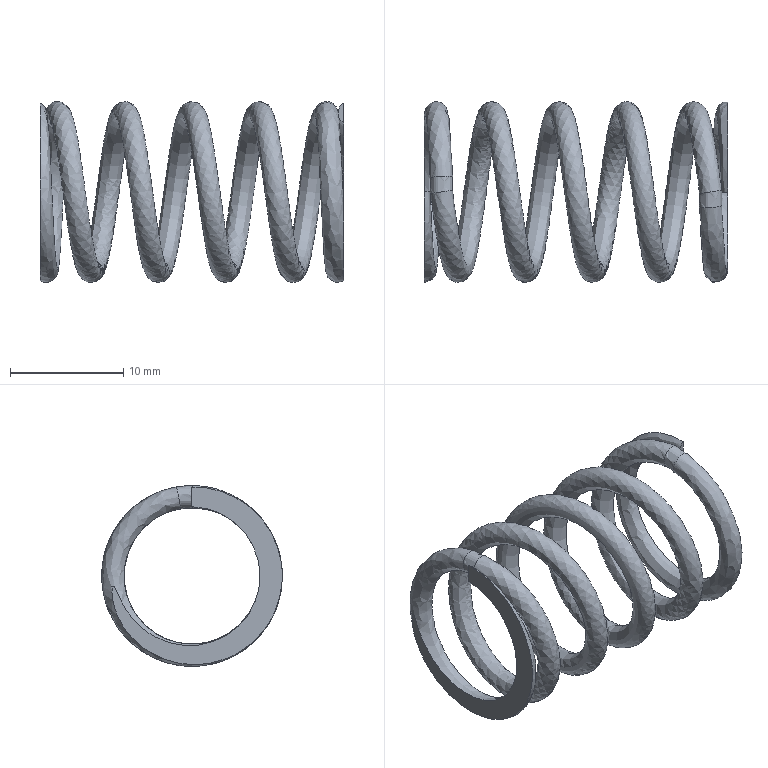Component | NX | VALVE_PORT_SPRING | 1 solid | 9 faces | volume 773 mm3 | spline 5 | plane 4